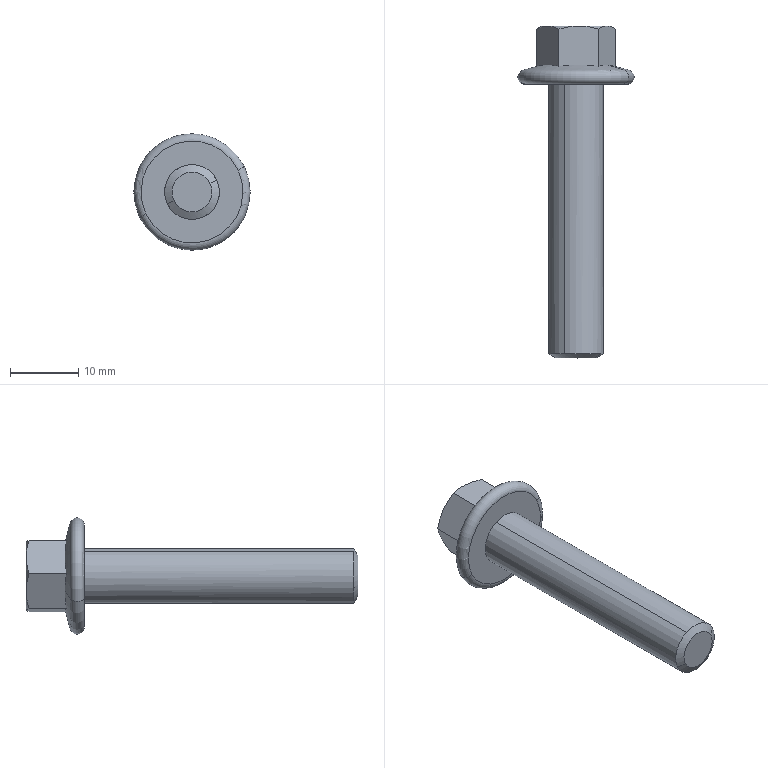Component | SolidWorks | GB_T16674-1996HexagonHeadFlangeBolt(SmallSeries)M8_40-2 | 1 solid | 27 faces | box 17 x 48.5 x 17 mm | volume 2950 mm3 | cone 11 | plane 10 | cylinder 4 | torus 2 | commonest cylinder face diameters 8.8 x2 8 x2
STEP:
#1=COLOUR_RGB('',0.7922,0.8196,0.9333);
#2=FILL_AREA_STYLE_COLOUR('',#1);
#3=FILL_AREA_STYLE('',(#2));
#4=SURFACE_STYLE_FILL_AREA(#3);
#5=SURFACE_SIDE_STYLE('',(#4));
#6=SURFACE_STYLE_USAGE(.BOTH.,#5);
#7=PRESENTATION_STYLE_ASSIGNMENT((#6));
#8=CARTESIAN_POINT('',(2.878,-0.7054,1.849));
#9=VERTEX_POINT('',#8);
#10=CARTESIAN_POINT('',(3.028,-0.7054,1.537));
#11=VERTEX_POINT('',#10);
#12=CARTESIAN_POINT('',(2.953,-0.7054,1.693));
#13=DIRECTION('',(0.,1.,0.));
#14=DIRECTION('',(0.4334,0.,-0.9012));
#15=AXIS2_PLACEMENT_3D('',#12,#13,#14);
#16=CIRCLE('',#15,0.1732);
#17=EDGE_CURVE('',#9,#11,#16,.T.);
#18=ORIENTED_EDGE('',*,*,#17,.F.);
#19=CARTESIAN_POINT('',(2.878,-0.6496,1.849));
#20=VERTEX_POINT('',#19);
#21=CARTESIAN_POINT('',(2.878,-0.7054,1.849));
#22=DIRECTION('',(0.,1.,0.));
#23=VECTOR('',#22,39.37);
#24=LINE('',#21,#23);
#25=EDGE_CURVE('',#9,#20,#24,.T.);
#26=ORIENTED_EDGE('',*,*,#25,.T.);
#27=CARTESIAN_POINT('',(3.028,-0.6496,1.537));
#28=VERTEX_POINT('',#27);
#29=CARTESIAN_POINT('',(2.953,-0.6496,1.693));
#30=DIRECTION('',(0.,1.,0.));
#31=DIRECTION('',(0.4334,0.,-0.9012));
#32=AXIS2_PLACEMENT_3D('',#29,#30,#31);
#33=CIRCLE('',#32,0.1732);
#34=EDGE_CURVE('',#20,#28,#33,.T.);
#35=ORIENTED_EDGE('',*,*,#34,.T.);
#36=CARTESIAN_POINT('',(3.028,-0.7054,1.537));
#37=DIRECTION('',(0.,1.,0.));
#38=VECTOR('',#37,39.37);
#39=LINE('',#36,#38);
#40=EDGE_CURVE('',#11,#28,#39,.T.);
#41=ORIENTED_EDGE('',*,*,#40,.F.);
#42=EDGE_LOOP('',(#18,#26,#35,#41));
#43=FACE_OUTER_BOUND('',#42,.T.);
#44=CARTESIAN_POINT('',(2.953,-0.7054,1.693));
#45=DIRECTION('',(0.,1.,0.));
#46=DIRECTION('',(0.4334,0.,-0.9012));
#47=AXIS2_PLACEMENT_3D('',#44,#45,#46);
#48=CYLINDRICAL_SURFACE('',#47,0.1732);
#49=ADVANCED_FACE('',(#43),#48,.F.);
#50=CARTESIAN_POINT('',(2.849,-2.559,1.643));
#51=VERTEX_POINT('',#50);
#52=CARTESIAN_POINT('',(3.056,-2.559,1.743));
#53=VERTEX_POINT('',#52);
#54=CARTESIAN_POINT('',(2.953,-2.559,1.693));
#55=DIRECTION('',(0.,-1.,0.));
#56=DIRECTION('',(-0.9012,0.,-0.4334));
#57=AXIS2_PLACEMENT_3D('',#54,#55,#56);
#58=CIRCLE('',#57,0.1149);
#59=EDGE_CURVE('',#51,#53,#58,.T.);
#60=ORIENTED_EDGE('',*,*,#59,.F.);
#61=CARTESIAN_POINT('',(2.811,-2.534,1.625));
#62=VERTEX_POINT('',#61);
#63=CARTESIAN_POINT('',(2.811,-2.534,1.625));
#64=DIRECTION('',(-0.7804,0.5,-0.3754));
#65=VECTOR('',#64,39.37);
#66=LINE('',#63,#65);
#67=EDGE_CURVE('',#51,#62,#66,.T.);
#68=ORIENTED_EDGE('',*,*,#67,.T.);
#69=CARTESIAN_POINT('',(3.021,-2.534,1.551));
#70=VERTEX_POINT('',#69);
#71=CARTESIAN_POINT('',(2.953,-2.534,1.693));
#72=DIRECTION('',(0.,-1.,0.));
#73=DIRECTION('',(-0.9012,0.,-0.4334));
#74=AXIS2_PLACEMENT_3D('',#71,#72,#73);
#75=CIRCLE('',#74,0.1575);
#76=EDGE_CURVE('',#62,#70,#75,.T.);
#77=ORIENTED_EDGE('',*,*,#76,.T.);
#78=CARTESIAN_POINT('',(3.095,-2.534,1.761));
#79=VERTEX_POINT('',#78);
#80=CARTESIAN_POINT('',(2.953,-2.534,1.693));
#81=DIRECTION('',(0.,-1.,0.));
#82=DIRECTION('',(-0.9012,0.,-0.4334));
#83=AXIS2_PLACEMENT_3D('',#80,#81,#82);
#84=CIRCLE('',#83,0.1575);
#85=EDGE_CURVE('',#70,#79,#84,.T.);
#86=ORIENTED_EDGE('',*,*,#85,.T.);
#87=CARTESIAN_POINT('',(3.095,-2.534,1.761));
#88=DIRECTION('',(0.7804,0.5,0.3754));
#89=VECTOR('',#88,39.37);
#90=LINE('',#87,#89);
#91=EDGE_CURVE('',#53,#79,#90,.T.);
#92=ORIENTED_EDGE('',*,*,#91,.F.);
#93=EDGE_LOOP('',(#60,#68,#77,#86,#92));
#94=FACE_OUTER_BOUND('',#93,.T.);
#95=CARTESIAN_POINT('',(2.953,-2.534,1.693));
#96=DIRECTION('',(0.,1.,0.));
#97=DIRECTION('',(0.9012,0.,0.4334));
#98=AXIS2_PLACEMENT_3D('',#95,#96,#97);
#99=CONICAL_SURFACE('',#98,0.1575,1.047);
#100=ADVANCED_FACE('',(#94),#99,.T.);
#101=CARTESIAN_POINT('',(2.884,-2.534,1.835));
#102=VERTEX_POINT('',#101);
#103=CARTESIAN_POINT('',(2.953,-2.534,1.693));
#104=DIRECTION('',(0.,-1.,0.));
#105=DIRECTION('',(-0.9012,0.,-0.4334));
#106=AXIS2_PLACEMENT_3D('',#103,#104,#105);
#107=CIRCLE('',#106,0.1575);
#108=EDGE_CURVE('',#102,#62,#107,.T.);
#109=ORIENTED_EDGE('',*,*,#108,.F.);
#110=CARTESIAN_POINT('',(2.884,-0.9843,1.835));
#111=VERTEX_POINT('',#110);
#112=CARTESIAN_POINT('',(2.884,-2.559,1.835));
#113=DIRECTION('',(0.,1.,0.));
#114=VECTOR('',#113,39.37);
#115=LINE('',#112,#114);
#116=EDGE_CURVE('',#102,#111,#115,.T.);
#117=ORIENTED_EDGE('',*,*,#116,.T.);
#118=CARTESIAN_POINT('',(3.021,-0.9843,1.551));
#119=VERTEX_POINT('',#118);
#120=CARTESIAN_POINT('',(2.953,-0.9843,1.693));
#121=DIRECTION('',(0.,-1.,0.));
#122=DIRECTION('',(0.4334,0.,-0.9012));
#123=AXIS2_PLACEMENT_3D('',#120,#121,#122);
#124=CIRCLE('',#123,0.1575);
#125=EDGE_CURVE('',#111,#119,#124,.T.);
#126=ORIENTED_EDGE('',*,*,#125,.T.);
#127=CARTESIAN_POINT('',(3.021,-2.559,1.551));
#128=DIRECTION('',(0.,1.,0.));
#129=VECTOR('',#128,39.37);
#130=LINE('',#127,#129);
#131=EDGE_CURVE('',#70,#119,#130,.T.);
#132=ORIENTED_EDGE('',*,*,#131,.F.);
#133=ORIENTED_EDGE('',*,*,#76,.F.);
#134=EDGE_LOOP('',(#109,#117,#126,#132,#133));
#135=FACE_OUTER_BOUND('',#134,.T.);
#136=CARTESIAN_POINT('',(2.953,-2.559,1.693));
#137=DIRECTION('',(0.,1.,0.));
#138=DIRECTION('',(0.4334,0.,-0.9012));
#139=AXIS2_PLACEMENT_3D('',#136,#137,#138);
#140=CYLINDRICAL_SURFACE('',#139,0.1575);
#141=ADVANCED_FACE('',(#135),#140,.T.);
#142=CARTESIAN_POINT('',(3.179,-0.8824,1.676));
#143=VERTEX_POINT('',#142);
#144=CARTESIAN_POINT('',(3.13,-0.8743,1.778));
#145=VERTEX_POINT('',#144);
#146=CARTESIAN_POINT('',(3.179,-0.8824,1.676));
#147=CARTESIAN_POINT('',(3.163,-0.8774,1.71));
#148=CARTESIAN_POINT('',(3.147,-0.8743,1.744));
#149=CARTESIAN_POINT('',(3.13,-0.8743,1.778));
#150=B_SPLINE_CURVE_WITH_KNOTS('',3,(#146,#147,#148,#149),.UNSPECIFIED.,.F.,.F.,(4,4),(0.,0.002894),.UNSPECIFIED.);
#151=EDGE_CURVE('',#143,#145,#150,.T.);
#152=ORIENTED_EDGE('',*,*,#151,.T.);
#153=CARTESIAN_POINT('',(3.227,-0.903,1.825));
#154=VERTEX_POINT('',#153);
#155=CARTESIAN_POINT('',(135.365,-40.192,65.378));
#156=DIRECTION('',(0.8705,-0.2588,0.4187));
#157=VECTOR('',#156,39.37);
#158=LINE('',#155,#157);
#159=EDGE_CURVE('',#145,#154,#158,.T.);
#160=ORIENTED_EDGE('',*,*,#159,.T.);
#161=CARTESIAN_POINT('',(2.679,-0.903,1.561));
#162=VERTEX_POINT('',#161);
#163=CARTESIAN_POINT('',(2.953,-0.903,1.693));
#164=DIRECTION('',(0.,1.,0.));
#165=DIRECTION('',(0.9012,0.,0.4334));
#166=AXIS2_PLACEMENT_3D('',#163,#164,#165);
#167=CIRCLE('',#166,0.304);
#168=EDGE_CURVE('',#154,#162,#167,.T.);
#169=ORIENTED_EDGE('',*,*,#168,.T.);
#170=CARTESIAN_POINT('',(2.775,-0.8743,1.608));
#171=VERTEX_POINT('',#170);
#172=CARTESIAN_POINT('',(-129.459,-40.192,-61.993));
#173=DIRECTION('',(-0.8705,-0.2588,-0.4187));
#174=VECTOR('',#173,39.37);
#175=LINE('',#172,#174);
#176=EDGE_CURVE('',#171,#162,#175,.T.);
#177=ORIENTED_EDGE('',*,*,#176,.F.);
#178=CARTESIAN_POINT('',(2.825,-0.8824,1.505));
#179=VERTEX_POINT('',#178);
#180=CARTESIAN_POINT('',(2.775,-0.8743,1.608));
#181=CARTESIAN_POINT('',(2.792,-0.8743,1.573));
#182=CARTESIAN_POINT('',(2.808,-0.8774,1.539));
#183=CARTESIAN_POINT('',(2.825,-0.8824,1.505));
#184=B_SPLINE_CURVE_WITH_KNOTS('',3,(#180,#181,#182,#183),.UNSPECIFIED.,.F.,.F.,(4,4),(-0.,0.002894),.UNSPECIFIED.);
#185=EDGE_CURVE('',#171,#179,#184,.T.);
#186=ORIENTED_EDGE('',*,*,#185,.T.);
#187=CARTESIAN_POINT('',(3.051,-0.8824,1.488));
#188=VERTEX_POINT('',#187);
#189=CARTESIAN_POINT('',(2.825,-0.8824,1.505));
#190=CARTESIAN_POINT('',(2.862,-0.8774,1.502));
#191=CARTESIAN_POINT('',(2.938,-0.8712,1.497));
#192=CARTESIAN_POINT('',(3.014,-0.8774,1.491));
#193=CARTESIAN_POINT('',(3.051,-0.8824,1.488));
#194=B_SPLINE_CURVE_WITH_KNOTS('',3,(#189,#190,#191,#192,#193),.UNSPECIFIED.,.F.,.F.,(4,1,4),(0.,0.002887,0.005774),.UNSPECIFIED.);
#195=EDGE_CURVE('',#179,#188,#194,.T.);
#196=ORIENTED_EDGE('',*,*,#195,.T.);
#197=CARTESIAN_POINT('',(3.051,-0.8824,1.488));
#198=CARTESIAN_POINT('',(3.073,-0.8774,1.519));
#199=CARTESIAN_POINT('',(3.115,-0.8712,1.582));
#200=CARTESIAN_POINT('',(3.158,-0.8774,1.645));
#201=CARTESIAN_POINT('',(3.179,-0.8824,1.676));
#202=B_SPLINE_CURVE_WITH_KNOTS('',3,(#197,#198,#199,#200,#201),.UNSPECIFIED.,.F.,.F.,(4,1,4),(0.,0.002887,0.005774),.UNSPECIFIED.);
#203=EDGE_CURVE('',#188,#143,#202,.T.);
#204=ORIENTED_EDGE('',*,*,#203,.T.);
#205=EDGE_LOOP('',(#152,#160,#169,#177,#186,#196,#204));
#206=FACE_OUTER_BOUND('',#205,.T.);
#207=CARTESIAN_POINT('',(2.953,-40.192,1.693));
#208=DIRECTION('',(0.,-1.,0.));
#209=DIRECTION('',(-0.9012,0.,-0.4334));
#210=AXIS2_PLACEMENT_3D('',#207,#208,#209);
#211=CONICAL_SURFACE('',#210,146.931,1.309);
#212=ADVANCED_FACE('',(#206),#211,.T.);
#213=CARTESIAN_POINT('',(3.217,-0.9843,1.82));
#214=VERTEX_POINT('',#213);
#215=CARTESIAN_POINT('',(2.688,-0.9843,1.566));
#216=VERTEX_POINT('',#215);
#217=CARTESIAN_POINT('',(2.953,-0.9843,1.693));
#218=DIRECTION('',(0.,1.,0.));
#219=DIRECTION('',(0.9012,0.,0.4334));
#220=AXIS2_PLACEMENT_3D('',#217,#218,#219);
#221=CIRCLE('',#220,0.2933);
#222=EDGE_CURVE('',#214,#216,#221,.T.);
#223=ORIENTED_EDGE('',*,*,#222,.T.);
#224=CARTESIAN_POINT('',(2.688,-0.9429,1.566));
#225=DIRECTION('',(0.4334,0.,-0.9012));
#226=DIRECTION('',(-0.9012,0.,-0.4334));
#227=AXIS2_PLACEMENT_3D('',#224,#225,#226);
#228=CIRCLE('',#227,0.04134);
#229=EDGE_CURVE('',#216,#162,#228,.T.);
#230=ORIENTED_EDGE('',*,*,#229,.T.);
#231=ORIENTED_EDGE('',*,*,#168,.F.);
#232=CARTESIAN_POINT('',(3.217,-0.9429,1.82));
#233=DIRECTION('',(-0.4334,0.,0.9012));
#234=DIRECTION('',(0.9012,0.,0.4334));
#235=AXIS2_PLACEMENT_3D('',#232,#233,#234);
#236=CIRCLE('',#235,0.04134);
#237=EDGE_CURVE('',#214,#154,#236,.T.);
#238=ORIENTED_EDGE('',*,*,#237,.F.);
#239=EDGE_LOOP('',(#223,#230,#231,#238));
#240=FACE_OUTER_BOUND('',#239,.T.);
#241=CARTESIAN_POINT('',(2.953,-0.9429,1.693));
#242=DIRECTION('',(-0.,1.,-0.));
#243=DIRECTION('',(0.9012,0.,0.4334));
#244=AXIS2_PLACEMENT_3D('',#241,#242,#243);
#245=TOROIDAL_SURFACE('',#244,0.2933,0.04134);
#246=ADVANCED_FACE('',(#240),#245,.T.);
#247=CARTESIAN_POINT('',(3.038,-0.6496,1.516));
#248=VERTEX_POINT('',#247);
#249=CARTESIAN_POINT('',(2.938,-0.6496,1.497));
#250=VERTEX_POINT('',#249);
#251=CARTESIAN_POINT('',(2.953,-0.6496,1.693));
#252=DIRECTION('',(0.,1.,0.));
#253=DIRECTION('',(0.4334,0.,-0.9012));
#254=AXIS2_PLACEMENT_3D('',#251,#252,#253);
#255=CIRCLE('',#254,0.1969);
#256=EDGE_CURVE('',#248,#250,#255,.T.);
#257=ORIENTED_EDGE('',*,*,#256,.F.);
#258=CARTESIAN_POINT('',(3.051,-0.6672,1.488));
#259=VERTEX_POINT('',#258);
#260=CARTESIAN_POINT('',(3.038,-0.6496,1.516));
#261=DIRECTION('',(0.3754,-0.5,-0.7804));
#262=VECTOR('',#261,39.37);
#263=LINE('',#260,#262);
#264=EDGE_CURVE('',#248,#259,#263,.T.);
#265=ORIENTED_EDGE('',*,*,#264,.T.);
#266=CARTESIAN_POINT('',(2.938,-0.6496,1.497));
#267=CARTESIAN_POINT('',(2.977,-0.6496,1.494));
#268=CARTESIAN_POINT('',(3.014,-0.6565,1.491));
#269=CARTESIAN_POINT('',(3.051,-0.6672,1.488));
#270=B_SPLINE_CURVE_WITH_KNOTS('',3,(#266,#267,#268,#269),.UNSPECIFIED.,.F.,.F.,(4,4),(0.,0.002921),.UNSPECIFIED.);
#271=EDGE_CURVE('',#250,#259,#270,.T.);
#272=ORIENTED_EDGE('',*,*,#271,.F.);
#273=EDGE_LOOP('',(#257,#265,#272));
#274=FACE_OUTER_BOUND('',#273,.T.);
#275=CARTESIAN_POINT('',(2.953,-0.6496,1.693));
#276=DIRECTION('',(0.,-1.,0.));
#277=DIRECTION('',(0.4334,0.,-0.9012));
#278=AXIS2_PLACEMENT_3D('',#275,#276,#277);
#279=CONICAL_SURFACE('',#278,0.1969,1.047);
#280=ADVANCED_FACE('',(#274),#279,.T.);
#281=CARTESIAN_POINT('',(2.953,-0.7054,1.693));
#282=DIRECTION('',(0.,1.,0.));
#283=DIRECTION('',(0.4334,0.,-0.9012));
#284=AXIS2_PLACEMENT_3D('',#281,#282,#283);
#285=CIRCLE('',#284,0.1732);
#286=EDGE_CURVE('',#11,#9,#285,.T.);
#287=ORIENTED_EDGE('',*,*,#286,.T.);
#288=ORIENTED_EDGE('',*,*,#17,.T.);
#289=EDGE_LOOP('',(#287,#288));
#290=FACE_OUTER_BOUND('',#289,.T.);
#291=CARTESIAN_POINT('',(2.953,-0.7054,1.693));
#292=DIRECTION('',(0.,1.,0.));
#293=DIRECTION('',(0.4334,0.,-0.9012));
#294=AXIS2_PLACEMENT_3D('',#291,#292,#293);
#295=PLANE('',#294);
#296=ADVANCED_FACE('',(#290),#295,.T.);
#297=CARTESIAN_POINT('',(2.953,-2.559,1.693));
#298=DIRECTION('',(0.,-1.,0.));
#299=DIRECTION('',(-0.9012,0.,-0.4334));
#300=AXIS2_PLACEMENT_3D('',#297,#298,#299);
#301=CIRCLE('',#300,0.1149);
#302=EDGE_CURVE('',#53,#51,#301,.T.);
#303=ORIENTED_EDGE('',*,*,#302,.T.);
#304=ORIENTED_EDGE('',*,*,#59,.T.);
#305=EDGE_LOOP('',(#303,#304));
#306=FACE_OUTER_BOUND('',#305,.T.);
#307=CARTESIAN_POINT('',(2.953,-2.559,1.693));
#308=DIRECTION('',(0.,-1.,0.));
#309=DIRECTION('',(0.9012,0.,0.4334));
#310=AXIS2_PLACEMENT_3D('',#307,#308,#309);
#311=PLANE('',#310);
#312=ADVANCED_FACE('',(#306),#311,.T.);
#313=CARTESIAN_POINT('',(2.953,-0.6496,1.693));
#314=DIRECTION('',(0.,1.,0.));
#315=DIRECTION('',(0.4334,0.,-0.9012));
#316=AXIS2_PLACEMENT_3D('',#313,#314,#315);
#317=CIRCLE('',#316,0.1732);
#318=EDGE_CURVE('',#28,#20,#317,.T.);
#319=ORIENTED_EDGE('',*,*,#318,.F.);
#320=ORIENTED_EDGE('',*,*,#34,.F.);
#321=EDGE_LOOP('',(#319,#320));
#322=FACE_BOUND('',#321,.T.);
#323=CARTESIAN_POINT('',(3.13,-0.6496,1.778));
#324=VERTEX_POINT('',#323);
#325=CARTESIAN_POINT('',(3.115,-0.6496,1.582));
#326=VERTEX_POINT('',#325);
#327=CARTESIAN_POINT('',(2.953,-0.6496,1.693));
#328=DIRECTION('',(0.,1.,0.));
#329=DIRECTION('',(0.4334,0.,-0.9012));
#330=AXIS2_PLACEMENT_3D('',#327,#328,#329);
#331=CIRCLE('',#330,0.1969);
#332=EDGE_CURVE('',#324,#326,#331,.T.);
#333=ORIENTED_EDGE('',*,*,#332,.T.);
#334=CARTESIAN_POINT('',(2.953,-0.6496,1.693));
#335=DIRECTION('',(0.,1.,0.));
#336=DIRECTION('',(0.4334,0.,-0.9012));
#337=AXIS2_PLACEMENT_3D('',#334,#335,#336);
#338=CIRCLE('',#337,0.1969);
#339=EDGE_CURVE('',#326,#248,#338,.T.);
#340=ORIENTED_EDGE('',*,*,#339,.T.);
#341=ORIENTED_EDGE('',*,*,#256,.T.);
#342=CARTESIAN_POINT('',(2.775,-0.6496,1.608));
#343=VERTEX_POINT('',#342);
#344=CARTESIAN_POINT('',(2.953,-0.6496,1.693));
#345=DIRECTION('',(0.,1.,0.));
#346=DIRECTION('',(0.4334,0.,-0.9012));
#347=AXIS2_PLACEMENT_3D('',#344,#345,#346);
#348=CIRCLE('',#347,0.1969);
#349=EDGE_CURVE('',#250,#343,#348,.T.);
#350=ORIENTED_EDGE('',*,*,#349,.T.);
#351=CARTESIAN_POINT('',(2.79,-0.6496,1.804));
#352=VERTEX_POINT('',#351);
#353=CARTESIAN_POINT('',(2.953,-0.6496,1.693));
#354=DIRECTION('',(0.,1.,0.));
#355=DIRECTION('',(0.4334,0.,-0.9012));
#356=AXIS2_PLACEMENT_3D('',#353,#354,#355);
#357=CIRCLE('',#356,0.1969);
#358=EDGE_CURVE('',#343,#352,#357,.T.);
#359=ORIENTED_EDGE('',*,*,#358,.T.);
#360=CARTESIAN_POINT('',(2.968,-0.6496,1.889));
#361=VERTEX_POINT('',#360);
#362=CARTESIAN_POINT('',(2.953,-0.6496,1.693));
#363=DIRECTION('',(0.,1.,0.));
#364=DIRECTION('',(0.4334,0.,-0.9012));
#365=AXIS2_PLACEMENT_3D('',#362,#363,#364);
#366=CIRCLE('',#365,0.1969);
#367=EDGE_CURVE('',#352,#361,#366,.T.);
#368=ORIENTED_EDGE('',*,*,#367,.T.);
#369=CARTESIAN_POINT('',(2.953,-0.6496,1.693));
#370=DIRECTION('',(0.,1.,0.));
#371=DIRECTION('',(0.4334,0.,-0.9012));
#372=AXIS2_PLACEMENT_3D('',#369,#370,#371);
#373=CIRCLE('',#372,0.1969);
#374=EDGE_CURVE('',#361,#324,#373,.T.);
#375=ORIENTED_EDGE('',*,*,#374,.T.);
#376=EDGE_LOOP('',(#333,#340,#341,#350,#359,#368,#375));
#377=FACE_OUTER_BOUND('',#376,.T.);
#378=CARTESIAN_POINT('',(3.051,-0.6496,1.488));
#379=DIRECTION('',(0.,1.,0.));
#380=DIRECTION('',(0.4334,0.,-0.9012));
#381=AXIS2_PLACEMENT_3D('',#378,#379,#380);
#382=PLANE('',#381);
#383=ADVANCED_FACE('',(#322,#377),#382,.T.);
#384=ORIENTED_EDGE('',*,*,#349,.F.);
#385=CARTESIAN_POINT('',(2.825,-0.6672,1.505));
#386=VERTEX_POINT('',#385);
#387=CARTESIAN_POINT('',(2.825,-0.6672,1.505));
#388=CARTESIAN_POINT('',(2.862,-0.6565,1.502));
#389=CARTESIAN_POINT('',(2.899,-0.6496,1.5));
#390=CARTESIAN_POINT('',(2.938,-0.6496,1.497));
#391=B_SPLINE_CURVE_WITH_KNOTS('',3,(#387,#388,#389,#390),.UNSPECIFIED.,.F.,.F.,(4,4),(0.,0.002921),.UNSPECIFIED.);
#392=EDGE_CURVE('',#386,#250,#391,.T.);
#393=ORIENTED_EDGE('',*,*,#392,.F.);
#394=CARTESIAN_POINT('',(2.775,-0.6496,1.608));
#395=CARTESIAN_POINT('',(2.792,-0.6496,1.573));
#396=CARTESIAN_POINT('',(2.809,-0.6565,1.539));
#397=CARTESIAN_POINT('',(2.825,-0.6672,1.505));
#398=B_SPLINE_CURVE_WITH_KNOTS('',3,(#394,#395,#396,#397),.UNSPECIFIED.,.F.,.F.,(4,4),(0.,0.002921),.UNSPECIFIED.);
#399=EDGE_CURVE('',#343,#386,#398,.T.);
#400=ORIENTED_EDGE('',*,*,#399,.F.);
#401=EDGE_LOOP('',(#384,#393,#400));
#402=FACE_OUTER_BOUND('',#401,.T.);
#403=CARTESIAN_POINT('',(2.953,-0.6496,1.693));
#404=DIRECTION('',(0.,-1.,0.));
#405=DIRECTION('',(0.4334,0.,-0.9012));
#406=AXIS2_PLACEMENT_3D('',#403,#404,#405);
#407=CONICAL_SURFACE('',#406,0.1969,1.047);
#408=ADVANCED_FACE('',(#402),#407,.T.);
#409=ORIENTED_EDGE('',*,*,#358,.F.);
#410=CARTESIAN_POINT('',(2.726,-0.6672,1.71));
#411=VERTEX_POINT('',#410);
#412=CARTESIAN_POINT('',(2.726,-0.6672,1.71));
#413=CARTESIAN_POINT('',(2.742,-0.6565,1.677));
#414=CARTESIAN_POINT('',(2.759,-0.6496,1.643));
#415=CARTESIAN_POINT('',(2.775,-0.6496,1.608));
#416=B_SPLINE_CURVE_WITH_KNOTS('',3,(#412,#413,#414,#415),.UNSPECIFIED.,.F.,.F.,(4,4),(0.,0.002921),.UNSPECIFIED.);
#417=EDGE_CURVE('',#411,#343,#416,.T.);
#418=ORIENTED_EDGE('',*,*,#417,.F.);
#419=CARTESIAN_POINT('',(2.79,-0.6496,1.804));
#420=CARTESIAN_POINT('',(2.768,-0.6496,1.772));
#421=CARTESIAN_POINT('',(2.747,-0.6565,1.741));
#422=CARTESIAN_POINT('',(2.726,-0.6672,1.71));
#423=B_SPLINE_CURVE_WITH_KNOTS('',3,(#419,#420,#421,#422),.UNSPECIFIED.,.F.,.F.,(4,4),(0.,0.002921),.UNSPECIFIED.);
#424=EDGE_CURVE('',#352,#411,#423,.T.);
#425=ORIENTED_EDGE('',*,*,#424,.F.);
#426=EDGE_LOOP('',(#409,#418,#425));
#427=FACE_OUTER_BOUND('',#426,.T.);
#428=CARTESIAN_POINT('',(2.953,-0.6496,1.693));
#429=DIRECTION('',(0.,-1.,0.));
#430=DIRECTION('',(0.4334,0.,-0.9012));
#431=AXIS2_PLACEMENT_3D('',#428,#429,#430);
#432=CONICAL_SURFACE('',#431,0.1969,1.047);
#433=ADVANCED_FACE('',(#427),#432,.T.);
#434=ORIENTED_EDGE('',*,*,#367,.F.);
#435=CARTESIAN_POINT('',(2.854,-0.6672,1.898));
#436=VERTEX_POINT('',#435);
#437=CARTESIAN_POINT('',(2.854,-0.6672,1.898));
#438=CARTESIAN_POINT('',(2.833,-0.6565,1.867));
#439=CARTESIAN_POINT('',(2.812,-0.6496,1.836));
#440=CARTESIAN_POINT('',(2.79,-0.6496,1.804));
#441=B_SPLINE_CURVE_WITH_KNOTS('',3,(#437,#438,#439,#440),.UNSPECIFIED.,.F.,.F.,(4,4),(0.,0.002921),.UNSPECIFIED.);
#442=EDGE_CURVE('',#436,#352,#441,.T.);
#443=ORIENTED_EDGE('',*,*,#442,.F.);
#444=CARTESIAN_POINT('',(2.968,-0.6496,1.889));
#445=CARTESIAN_POINT('',(2.929,-0.6496,1.892));
#446=CARTESIAN_POINT('',(2.891,-0.6565,1.895));
#447=CARTESIAN_POINT('',(2.854,-0.6672,1.898));
#448=B_SPLINE_CURVE_WITH_KNOTS('',3,(#444,#445,#446,#447),.UNSPECIFIED.,.F.,.F.,(4,4),(0.,0.002921),.UNSPECIFIED.);
#449=EDGE_CURVE('',#361,#436,#448,.T.);
#450=ORIENTED_EDGE('',*,*,#449,.F.);
#451=EDGE_LOOP('',(#434,#443,#450));
#452=FACE_OUTER_BOUND('',#451,.T.);
#453=CARTESIAN_POINT('',(2.953,-0.6496,1.693));
#454=DIRECTION('',(0.,-1.,0.));
#455=DIRECTION('',(0.4334,0.,-0.9012));
#456=AXIS2_PLACEMENT_3D('',#453,#454,#455);
#457=CONICAL_SURFACE('',#456,0.1969,1.047);
#458=ADVANCED_FACE('',(#452),#457,.T.);
#459=ORIENTED_EDGE('',*,*,#374,.F.);
#460=CARTESIAN_POINT('',(3.081,-0.6672,1.881));
#461=VERTEX_POINT('',#460);
#462=CARTESIAN_POINT('',(3.081,-0.6672,1.881));
#463=CARTESIAN_POINT('',(3.044,-0.6565,1.883));
#464=CARTESIAN_POINT('',(3.006,-0.6496,1.886));
#465=CARTESIAN_POINT('',(2.968,-0.6496,1.889));
#466=B_SPLINE_CURVE_WITH_KNOTS('',3,(#462,#463,#464,#465),.UNSPECIFIED.,.F.,.F.,(4,4),(0.,0.002921),.UNSPECIFIED.);
#467=EDGE_CURVE('',#461,#361,#466,.T.);
#468=ORIENTED_EDGE('',*,*,#467,.F.);
#469=CARTESIAN_POINT('',(3.13,-0.6496,1.778));
#470=CARTESIAN_POINT('',(3.113,-0.6496,1.813));
#471=CARTESIAN_POINT('',(3.097,-0.6565,1.847));
#472=CARTESIAN_POINT('',(3.081,-0.6672,1.881));
#473=B_SPLINE_CURVE_WITH_KNOTS('',3,(#469,#470,#471,#472),.UNSPECIFIED.,.F.,.F.,(4,4),(0.,0.002921),.UNSPECIFIED.);
#474=EDGE_CURVE('',#324,#461,#473,.T.);
#475=ORIENTED_EDGE('',*,*,#474,.F.);
#476=EDGE_LOOP('',(#459,#468,#475));
#477=FACE_OUTER_BOUND('',#476,.T.);
#478=CARTESIAN_POINT('',(2.953,-0.6496,1.693));
#479=DIRECTION('',(0.,-1.,0.));
#480=DIRECTION('',(0.4334,0.,-0.9012));
#481=AXIS2_PLACEMENT_3D('',#478,#479,#480);
#482=CONICAL_SURFACE('',#481,0.1969,1.047);
#483=ADVANCED_FACE('',(#477),#482,.T.);
#484=ORIENTED_EDGE('',*,*,#332,.F.);
#485=CARTESIAN_POINT('',(3.179,-0.6672,1.676));
#486=VERTEX_POINT('',#485);
#487=CARTESIAN_POINT('',(3.179,-0.6672,1.676));
#488=CARTESIAN_POINT('',(3.163,-0.6565,1.709));
#489=CARTESIAN_POINT('',(3.147,-0.6496,1.743));
#490=CARTESIAN_POINT('',(3.13,-0.6496,1.778));
#491=B_SPLINE_CURVE_WITH_KNOTS('',3,(#487,#488,#489,#490),.UNSPECIFIED.,.F.,.F.,(4,4),(0.,0.002921),.UNSPECIFIED.);
#492=EDGE_CURVE('',#486,#324,#491,.T.);
#493=ORIENTED_EDGE('',*,*,#492,.F.);
#494=CARTESIAN_POINT('',(3.115,-0.6496,1.582));
#495=CARTESIAN_POINT('',(3.137,-0.6496,1.614));
#496=CARTESIAN_POINT('',(3.158,-0.6565,1.645));
#497=CARTESIAN_POINT('',(3.179,-0.6672,1.676));
#498=B_SPLINE_CURVE_WITH_KNOTS('',3,(#494,#495,#496,#497),.UNSPECIFIED.,.F.,.F.,(4,4),(0.,0.002921),.UNSPECIFIED.);
#499=EDGE_CURVE('',#326,#486,#498,.T.);
#500=ORIENTED_EDGE('',*,*,#499,.F.);
#501=EDGE_LOOP('',(#484,#493,#500));
#502=FACE_OUTER_BOUND('',#501,.T.);
#503=CARTESIAN_POINT('',(2.953,-0.6496,1.693));
#504=DIRECTION('',(0.,-1.,0.));
#505=DIRECTION('',(0.4334,0.,-0.9012));
#506=AXIS2_PLACEMENT_3D('',#503,#504,#505);
#507=CONICAL_SURFACE('',#506,0.1969,1.047);
#508=ADVANCED_FACE('',(#502),#507,.T.);
#509=ORIENTED_EDGE('',*,*,#195,.F.);
#510=CARTESIAN_POINT('',(2.825,-0.9843,1.505));
#511=DIRECTION('',(0.,1.,0.));
#512=VECTOR('',#511,39.37);
#513=LINE('',#510,#512);
#514=EDGE_CURVE('',#179,#386,#513,.T.);
#515=ORIENTED_EDGE('',*,*,#514,.T.);
#516=ORIENTED_EDGE('',*,*,#392,.T.);
#517=ORIENTED_EDGE('',*,*,#271,.T.);
#518=CARTESIAN_POINT('',(3.051,-0.9843,1.488));
#519=DIRECTION('',(0.,1.,0.));
#520=VECTOR('',#519,39.37);
#521=LINE('',#518,#520);
#522=EDGE_CURVE('',#188,#259,#521,.T.);
#523=ORIENTED_EDGE('',*,*,#522,.F.);
#524=EDGE_LOOP('',(#509,#515,#516,#517,#523));
#525=FACE_OUTER_BOUND('',#524,.T.);
#526=CARTESIAN_POINT('',(3.051,-0.9843,1.488));
#527=DIRECTION('',(-0.07522,0.,-0.9972));
#528=DIRECTION('',(0.,-1.,0.));
#529=AXIS2_PLACEMENT_3D('',#526,#527,#528);
#530=PLANE('',#529);
#531=ADVANCED_FACE('',(#525),#530,.T.);
#532=CARTESIAN_POINT('',(2.726,-0.8824,1.71));
#533=VERTEX_POINT('',#532);
#534=CARTESIAN_POINT('',(2.726,-0.8824,1.71));
#535=CARTESIAN_POINT('',(2.742,-0.8774,1.676));
#536=CARTESIAN_POINT('',(2.759,-0.8743,1.642));
#537=CARTESIAN_POINT('',(2.775,-0.8743,1.608));
#538=B_SPLINE_CURVE_WITH_KNOTS('',3,(#534,#535,#536,#537),.UNSPECIFIED.,.F.,.F.,(4,4),(-0.002894,-0.),.UNSPECIFIED.);
#539=EDGE_CURVE('',#533,#171,#538,.T.);
#540=ORIENTED_EDGE('',*,*,#539,.F.);
#541=CARTESIAN_POINT('',(2.726,-0.9843,1.71));
#542=DIRECTION('',(0.,1.,0.));
#543=VECTOR('',#542,39.37);
#544=LINE('',#541,#543);
#545=EDGE_CURVE('',#533,#411,#544,.T.);
#546=ORIENTED_EDGE('',*,*,#545,.T.);
#547=ORIENTED_EDGE('',*,*,#417,.T.);
#548=ORIENTED_EDGE('',*,*,#399,.T.);
#549=ORIENTED_EDGE('',*,*,#514,.F.);
#550=ORIENTED_EDGE('',*,*,#185,.F.);
#551=EDGE_LOOP('',(#540,#546,#547,#548,#549,#550));
#552=FACE_OUTER_BOUND('',#551,.T.);
#553=CARTESIAN_POINT('',(2.825,-0.9843,1.505));
#554=DIRECTION('',(-0.9012,0.,-0.4334));
#555=DIRECTION('',(0.4334,0.,-0.9012));
#556=AXIS2_PLACEMENT_3D('',#553,#554,#555);
#557=PLANE('',#556);
#558=ADVANCED_FACE('',(#552),#557,.T.);
#559=CARTESIAN_POINT('',(2.854,-0.8824,1.898));
#560=VERTEX_POINT('',#559);
#561=CARTESIAN_POINT('',(2.854,-0.8824,1.898));
#562=CARTESIAN_POINT('',(2.833,-0.8774,1.866));
#563=CARTESIAN_POINT('',(2.79,-0.8712,1.804));
#564=CARTESIAN_POINT('',(2.747,-0.8774,1.741));
#565=CARTESIAN_POINT('',(2.726,-0.8824,1.71));
#566=B_SPLINE_CURVE_WITH_KNOTS('',3,(#561,#562,#563,#564,#565),.UNSPECIFIED.,.F.,.F.,(4,1,4),(0.,0.002887,0.005774),.UNSPECIFIED.);
#567=EDGE_CURVE('',#560,#533,#566,.T.);
#568=ORIENTED_EDGE('',*,*,#567,.F.);
#569=CARTESIAN_POINT('',(2.854,-0.9843,1.898));
#570=DIRECTION('',(0.,1.,0.));
#571=VECTOR('',#570,39.37);
#572=LINE('',#569,#571);
#573=EDGE_CURVE('',#560,#436,#572,.T.);
#574=ORIENTED_EDGE('',*,*,#573,.T.);
#575=ORIENTED_EDGE('',*,*,#442,.T.);
#576=ORIENTED_EDGE('',*,*,#424,.T.);
#577=ORIENTED_EDGE('',*,*,#545,.F.);
#578=EDGE_LOOP('',(#568,#574,#575,#576,#577));
#579=FACE_OUTER_BOUND('',#578,.T.);
#580=CARTESIAN_POINT('',(2.726,-0.9843,1.71));
#581=DIRECTION('',(-0.826,0.,0.5637));
#582=DIRECTION('',(0.,1.,0.));
#583=AXIS2_PLACEMENT_3D('',#580,#581,#582);
#584=PLANE('',#583);
#585=ADVANCED_FACE('',(#579),#584,.T.);
#586=CARTESIAN_POINT('',(3.081,-0.8824,1.881));
#587=VERTEX_POINT('',#586);
#588=CARTESIAN_POINT('',(3.081,-0.8824,1.881));
#589=CARTESIAN_POINT('',(3.043,-0.8774,1.884));
#590=CARTESIAN_POINT('',(2.968,-0.8712,1.889));
#591=CARTESIAN_POINT('',(2.892,-0.8774,1.895));
#592=CARTESIAN_POINT('',(2.854,-0.8824,1.898));
#593=B_SPLINE_CURVE_WITH_KNOTS('',3,(#588,#589,#590,#591,#592),.UNSPECIFIED.,.F.,.F.,(4,1,4),(0.,0.002887,0.005774),.UNSPECIFIED.);
#594=EDGE_CURVE('',#587,#560,#593,.T.);
#595=ORIENTED_EDGE('',*,*,#594,.F.);
#596=CARTESIAN_POINT('',(3.081,-0.9843,1.881));
#597=DIRECTION('',(0.,1.,0.));
#598=VECTOR('',#597,39.37);
#599=LINE('',#596,#598);
#600=EDGE_CURVE('',#587,#461,#599,.T.);
#601=ORIENTED_EDGE('',*,*,#600,.T.);
#602=ORIENTED_EDGE('',*,*,#467,.T.);
#603=ORIENTED_EDGE('',*,*,#449,.T.);
#604=ORIENTED_EDGE('',*,*,#573,.F.);
#605=EDGE_LOOP('',(#595,#601,#602,#603,#604));
#606=FACE_OUTER_BOUND('',#605,.T.);
#607=CARTESIAN_POINT('',(2.854,-0.9843,1.898));
#608=DIRECTION('',(0.07522,0.,0.9972));
#609=DIRECTION('',(-0.9972,0.,0.07522));
#610=AXIS2_PLACEMENT_3D('',#607,#608,#609);
#611=PLANE('',#610);
#612=ADVANCED_FACE('',(#606),#611,.T.);
#613=ORIENTED_EDGE('',*,*,#151,.F.);
#614=CARTESIAN_POINT('',(3.179,-0.9843,1.676));
#615=DIRECTION('',(0.,1.,0.));
#616=VECTOR('',#615,39.37);
#617=LINE('',#614,#616);
#618=EDGE_CURVE('',#143,#486,#617,.T.);
#619=ORIENTED_EDGE('',*,*,#618,.T.);
#620=ORIENTED_EDGE('',*,*,#492,.T.);
#621=ORIENTED_EDGE('',*,*,#474,.T.);
#622=ORIENTED_EDGE('',*,*,#600,.F.);
#623=CARTESIAN_POINT('',(3.13,-0.8743,1.778));
#624=CARTESIAN_POINT('',(3.114,-0.8743,1.813));
#625=CARTESIAN_POINT('',(3.097,-0.8774,1.847));
#626=CARTESIAN_POINT('',(3.081,-0.8824,1.881));
#627=B_SPLINE_CURVE_WITH_KNOTS('',3,(#623,#624,#625,#626),.UNSPECIFIED.,.F.,.F.,(4,4),(0.002894,0.005788),.UNSPECIFIED.);
#628=EDGE_CURVE('',#145,#587,#627,.T.);
#629=ORIENTED_EDGE('',*,*,#628,.F.);
#630=EDGE_LOOP('',(#613,#619,#620,#621,#622,#629));
#631=FACE_OUTER_BOUND('',#630,.T.);
#632=CARTESIAN_POINT('',(3.081,-0.9843,1.881));
#633=DIRECTION('',(0.9012,0.,0.4334));
#634=DIRECTION('',(0.,-1.,0.));
#635=AXIS2_PLACEMENT_3D('',#632,#633,#634);
#636=PLANE('',#635);
#637=ADVANCED_FACE('',(#631),#636,.T.);
#638=ORIENTED_EDGE('',*,*,#203,.F.);
#639=ORIENTED_EDGE('',*,*,#522,.T.);
#640=CARTESIAN_POINT('',(3.051,-0.6672,1.488));
#641=CARTESIAN_POINT('',(3.072,-0.6565,1.519));
#642=CARTESIAN_POINT('',(3.093,-0.6496,1.55));
#643=CARTESIAN_POINT('',(3.115,-0.6496,1.582));
#644=B_SPLINE_CURVE_WITH_KNOTS('',3,(#640,#641,#642,#643),.UNSPECIFIED.,.F.,.F.,(4,4),(0.,0.002921),.UNSPECIFIED.);
#645=EDGE_CURVE('',#259,#326,#644,.T.);
#646=ORIENTED_EDGE('',*,*,#645,.T.);
#647=ORIENTED_EDGE('',*,*,#499,.T.);
#648=ORIENTED_EDGE('',*,*,#618,.F.);
#649=EDGE_LOOP('',(#638,#639,#646,#647,#648));
#650=FACE_OUTER_BOUND('',#649,.T.);
#651=CARTESIAN_POINT('',(3.179,-0.9843,1.676));
#652=DIRECTION('',(0.826,0.,-0.5637));
#653=DIRECTION('',(0.,-1.,0.));
#654=AXIS2_PLACEMENT_3D('',#651,#652,#653);
#655=PLANE('',#654);
#656=ADVANCED_FACE('',(#650),#655,.T.);
#657=CARTESIAN_POINT('',(2.953,-0.9843,1.693));
#658=DIRECTION('',(0.,-1.,0.));
#659=DIRECTION('',(0.4334,0.,-0.9012));
#660=AXIS2_PLACEMENT_3D('',#657,#658,#659);
#661=CIRCLE('',#660,0.1575);
#662=EDGE_CURVE('',#119,#111,#661,.T.);
#663=ORIENTED_EDGE('',*,*,#662,.F.);
#664=ORIENTED_EDGE('',*,*,#125,.F.);
#665=EDGE_LOOP('',(#663,#664));
#666=FACE_BOUND('',#665,.T.);
#667=ORIENTED_EDGE('',*,*,#222,.F.);
#668=CARTESIAN_POINT('',(2.953,-0.9843,1.693));
#669=DIRECTION('',(0.,1.,0.));
#670=DIRECTION('',(0.9012,0.,0.4334));
#671=AXIS2_PLACEMENT_3D('',#668,#669,#670);
#672=CIRCLE('',#671,0.2933);
#673=EDGE_CURVE('',#216,#214,#672,.T.);
#674=ORIENTED_EDGE('',*,*,#673,.F.);
#675=EDGE_LOOP('',(#667,#674));
#676=FACE_OUTER_BOUND('',#675,.T.);
#677=CARTESIAN_POINT('',(3.051,-0.9843,1.488));
#678=DIRECTION('',(0.,1.,0.));
#679=DIRECTION('',(0.4334,0.,-0.9012));
#680=AXIS2_PLACEMENT_3D('',#677,#678,#679);
#681=PLANE('',#680);
#682=ADVANCED_FACE('',(#666,#676),#681,.F.);
#683=ORIENTED_EDGE('',*,*,#264,.F.);
#684=ORIENTED_EDGE('',*,*,#339,.F.);
#685=ORIENTED_EDGE('',*,*,#645,.F.);
#686=EDGE_LOOP('',(#683,#684,#685));
#687=FACE_OUTER_BOUND('',#686,.T.);
#688=CARTESIAN_POINT('',(2.953,-0.6496,1.693));
#689=DIRECTION('',(0.,-1.,0.));
#690=DIRECTION('',(0.4334,0.,-0.9012));
#691=AXIS2_PLACEMENT_3D('',#688,#689,#690);
#692=CONICAL_SURFACE('',#691,0.1969,1.047);
#693=ADVANCED_FACE('',(#687),#692,.T.);
#694=ORIENTED_EDGE('',*,*,#229,.F.);
#695=ORIENTED_EDGE('',*,*,#673,.T.);
#696=ORIENTED_EDGE('',*,*,#237,.T.);
#697=CARTESIAN_POINT('',(2.953,-0.903,1.693));
#698=DIRECTION('',(0.,1.,0.));
#699=DIRECTION('',(0.9012,0.,0.4334));
#700=AXIS2_PLACEMENT_3D('',#697,#698,#699);
#701=CIRCLE('',#700,0.304);
#702=EDGE_CURVE('',#162,#154,#701,.T.);
#703=ORIENTED_EDGE('',*,*,#702,.F.);
#704=EDGE_LOOP('',(#694,#695,#696,#703));
#705=FACE_OUTER_BOUND('',#704,.T.);
#706=CARTESIAN_POINT('',(2.953,-0.9429,1.693));
#707=DIRECTION('',(-0.,1.,-0.));
#708=DIRECTION('',(0.9012,0.,0.4334));
#709=AXIS2_PLACEMENT_3D('',#706,#707,#708);
#710=TOROIDAL_SURFACE('',#709,0.2933,0.04134);
#711=ADVANCED_FACE('',(#705),#710,.T.);
#712=ORIENTED_EDGE('',*,*,#159,.F.);
#713=ORIENTED_EDGE('',*,*,#628,.T.);
#714=ORIENTED_EDGE('',*,*,#594,.T.);
#715=ORIENTED_EDGE('',*,*,#567,.T.);
#716=ORIENTED_EDGE('',*,*,#539,.T.);
#717=ORIENTED_EDGE('',*,*,#176,.T.);
#718=ORIENTED_EDGE('',*,*,#702,.T.);
#719=EDGE_LOOP('',(#712,#713,#714,#715,#716,#717,#718));
#720=FACE_OUTER_BOUND('',#719,.T.);
#721=CARTESIAN_POINT('',(2.953,-40.192,1.693));
#722=DIRECTION('',(0.,-1.,0.));
#723=DIRECTION('',(-0.9012,0.,-0.4334));
#724=AXIS2_PLACEMENT_3D('',#721,#722,#723);
#725=CONICAL_SURFACE('',#724,146.931,1.309);
#726=ADVANCED_FACE('',(#720),#725,.T.);
#727=ORIENTED_EDGE('',*,*,#116,.F.);
#728=CARTESIAN_POINT('',(2.953,-2.534,1.693));
#729=DIRECTION('',(0.,-1.,0.));
#730=DIRECTION('',(-0.9012,0.,-0.4334));
#731=AXIS2_PLACEMENT_3D('',#728,#729,#730);
#732=CIRCLE('',#731,0.1575);
#733=EDGE_CURVE('',#79,#102,#732,.T.);
#734=ORIENTED_EDGE('',*,*,#733,.F.);
#735=ORIENTED_EDGE('',*,*,#85,.F.);
#736=ORIENTED_EDGE('',*,*,#131,.T.);
#737=ORIENTED_EDGE('',*,*,#662,.T.);
#738=EDGE_LOOP('',(#727,#734,#735,#736,#737));
#739=FACE_OUTER_BOUND('',#738,.T.);
#740=CARTESIAN_POINT('',(2.953,-2.559,1.693));
#741=DIRECTION('',(0.,1.,0.));
#742=DIRECTION('',(0.4334,0.,-0.9012));
#743=AXIS2_PLACEMENT_3D('',#740,#741,#742);
#744=CYLINDRICAL_SURFACE('',#743,0.1575);
#745=ADVANCED_FACE('',(#739),#744,.T.);
#746=ORIENTED_EDGE('',*,*,#67,.F.);
#747=ORIENTED_EDGE('',*,*,#302,.F.);
#748=ORIENTED_EDGE('',*,*,#91,.T.);
#749=ORIENTED_EDGE('',*,*,#733,.T.);
#750=ORIENTED_EDGE('',*,*,#108,.T.);
#751=EDGE_LOOP('',(#746,#747,#748,#749,#750));
#752=FACE_OUTER_BOUND('',#751,.T.);
#753=CARTESIAN_POINT('',(2.953,-2.534,1.693));
#754=DIRECTION('',(0.,1.,0.));
#755=DIRECTION('',(0.9012,0.,0.4334));
#756=AXIS2_PLACEMENT_3D('',#753,#754,#755);
#757=CONICAL_SURFACE('',#756,0.1575,1.047);
#758=ADVANCED_FACE('',(#752),#757,.T.);
#759=ORIENTED_EDGE('',*,*,#25,.F.);
#760=ORIENTED_EDGE('',*,*,#286,.F.);
#761=ORIENTED_EDGE('',*,*,#40,.T.);
#762=ORIENTED_EDGE('',*,*,#318,.T.);
#763=EDGE_LOOP('',(#759,#760,#761,#762));
#764=FACE_OUTER_BOUND('',#763,.T.);
#765=CARTESIAN_POINT('',(2.953,-0.7054,1.693));
#766=DIRECTION('',(0.,1.,0.));
#767=DIRECTION('',(0.4334,0.,-0.9012));
#768=AXIS2_PLACEMENT_3D('',#765,#766,#767);
#769=CYLINDRICAL_SURFACE('',#768,0.1732);
#770=ADVANCED_FACE('',(#764),#769,.F.);
#771=CLOSED_SHELL('',(#49,#100,#141,#212,#246,#280,#296,#312,#383,#408,#433,#458,#483,#508,#531,#558,#585,#612,#637,#656,#682,#693,#711,#726,#745,#758,#770));
#772=MANIFOLD_SOLID_BREP('',#771);
#773=STYLED_ITEM('',(#7),#772);
#774=(LENGTH_UNIT()NAMED_UNIT(*)SI_UNIT($,.METRE.));
#775=LENGTH_MEASURE_WITH_UNIT(LENGTH_MEASURE(0.0254),#774);
#776=DIMENSIONAL_EXPONENTS(1.,0.,0.,0.,0.,0.,0.);
#777=(CONVERSION_BASED_UNIT('',#775)LENGTH_UNIT()NAMED_UNIT(#776));
#778=UNCERTAINTY_MEASURE_WITH_UNIT(LENGTH_MEASURE(0.00001),#777,'','');
#779=(NAMED_UNIT(*)PLANE_ANGLE_UNIT()SI_UNIT($,.RADIAN.));
#780=(NAMED_UNIT(*)SI_UNIT($,.STERADIAN.)SOLID_ANGLE_UNIT());
#781=(GEOMETRIC_REPRESENTATION_CONTEXT(3)GLOBAL_UNCERTAINTY_ASSIGNED_CONTEXT((#778))GLOBAL_UNIT_ASSIGNED_CONTEXT((#777,#779,#780))REPRESENTATION_CONTEXT('',''));
#782=MECHANICAL_DESIGN_GEOMETRIC_PRESENTATION_REPRESENTATION('',(#773),#781);
#783=PRESENTATION_LAYER_ASSIGNMENT('','',(#773));
#784=CARTESIAN_POINT('',(0.,0.,0.));
#785=DIRECTION('',(0.,0.,1.));
#786=DIRECTION('',(1.,0.,0.));
#787=AXIS2_PLACEMENT_3D('',#784,#785,#786);
#788=(LENGTH_UNIT()NAMED_UNIT(*)SI_UNIT($,.METRE.));
#789=LENGTH_MEASURE_WITH_UNIT(LENGTH_MEASURE(0.0254),#788);
#790=DIMENSIONAL_EXPONENTS(1.,0.,0.,0.,0.,0.,0.);
#791=(CONVERSION_BASED_UNIT('',#789)LENGTH_UNIT()NAMED_UNIT(#790));
#792=UNCERTAINTY_MEASURE_WITH_UNIT(LENGTH_MEASURE(0.00001),#791,'','');
#793=(NAMED_UNIT(*)PLANE_ANGLE_UNIT()SI_UNIT($,.RADIAN.));
#794=(NAMED_UNIT(*)SI_UNIT($,.STERADIAN.)SOLID_ANGLE_UNIT());
#795=(GEOMETRIC_REPRESENTATION_CONTEXT(3)GLOBAL_UNCERTAINTY_ASSIGNED_CONTEXT((#792))GLOBAL_UNIT_ASSIGNED_CONTEXT((#791,#793,#794))REPRESENTATION_CONTEXT('',''));
#796=ADVANCED_BREP_SHAPE_REPRESENTATION('',(#772,#787),#795);